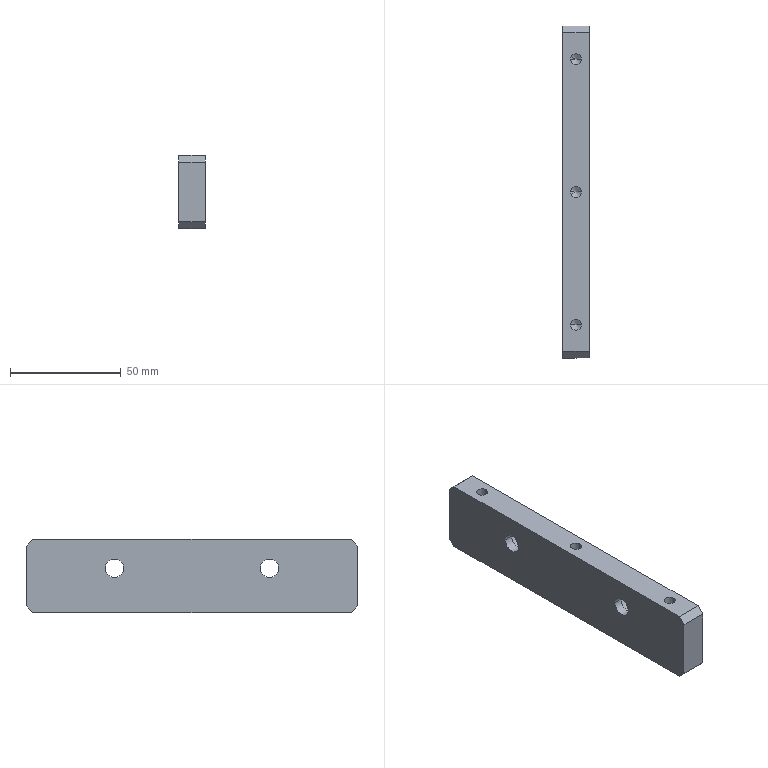Component | SolidWorks | A-C18EjectorMechanismConnectingBlock2-2 | 1 solid | 32 faces | box 12 x 150 x 33 mm | volume 55365 mm3 | cylinder 14 | plane 12 | cone 6 | commonest cylinder face diameters 5 x6 14 x4 8.4 x4
build123d program:
from build123d import *

# Parameters (mm, degrees)
SKETCH1_W                                       = 150
SKETCH1_H                                       = 33
BOSS_EXTRUDE1_DEPTH                             = 12
CHAMFER1_SIZE                                   = 3
M8_HEX_SOCKET_HEAD_CAP_SCREW_CBORE1_D           = 8.4
M8_HEX_SOCKET_HEAD_CAP_SCREW_CBORE1_CBORE_D     = 14
M8_HEX_SOCKET_HEAD_CAP_SCREW_CBORE1_CBORE_DEPTH = 8
M6_TAPPED_HOLE1_D                               = 5
M6_TAPPED_HOLE1_DEPTH                           = 15
M6_TAPPED_HOLE1_TIP                             = 1.502


with BuildPart() as part:
    # Sketch1 → Boss-Extrude1 (new body)
    with BuildSketch(Plane.XY):
        Rectangle(SKETCH1_W, SKETCH1_H)
    extrude(amount=BOSS_EXTRUDE1_DEPTH)

    # Chamfer1
    chamfer1_edges = [part.edges().sort_by_distance(p)[0] for p in [
        (75, -16.5, 6),
        (-75, -16.5, 6),
        (-75, 16.5, 6),
        (75, 16.5, 6),
    ]]
    chamfer(chamfer1_edges, length=CHAMFER1_SIZE)

    # M8 Hex Socket Head Cap Screw CBORE1 (through all)
    with Locations(Plane(origin=(0, 0, 0), x_dir=(-1, 0, 0), z_dir=(0, 0, -1))):
        with Locations((35, -3.5), (-35, -3.5)):
            CounterBoreHole(M8_HEX_SOCKET_HEAD_CAP_SCREW_CBORE1_D / 2, M8_HEX_SOCKET_HEAD_CAP_SCREW_CBORE1_CBORE_D / 2, M8_HEX_SOCKET_HEAD_CAP_SCREW_CBORE1_CBORE_DEPTH)

    # M6 Tapped Hole1
    with Locations(Plane.XZ.offset(16.5)):
        with Locations((-60, 6), (0, 6), (60, 6)):
            Hole(M6_TAPPED_HOLE1_D / 2, depth=M6_TAPPED_HOLE1_DEPTH)
            with Locations((0, 0, -(M6_TAPPED_HOLE1_DEPTH + M6_TAPPED_HOLE1_TIP / 2))):  # 118° drill point
                Cone(0, M6_TAPPED_HOLE1_D / 2, M6_TAPPED_HOLE1_TIP, mode=Mode.SUBTRACT)


solid = part.part

# Placed as in the assembly
solid = solid.moved(Location((-81.181, 22.568, -16.5), (-90, -90, 0)))
STEP:
#1=CARTESIAN_POINT('',(-3.531,-1.474,-0.5906));
#2=VERTEX_POINT('',#1);
#3=CARTESIAN_POINT('',(-3.334,-1.474,-0.5906));
#4=VERTEX_POINT('',#3);
#5=CARTESIAN_POINT('',(-3.432,-1.474,-0.5906));
#6=DIRECTION('',(0.,0.,1.));
#7=DIRECTION('',(1.,0.,0.));
#8=AXIS2_PLACEMENT_3D('',#5,#6,#7);
#9=CIRCLE('',#8,0.09843);
#10=EDGE_CURVE('',#2,#4,#9,.T.);
#11=ORIENTED_EDGE('',*,*,#10,.F.);
#12=CARTESIAN_POINT('',(-3.531,-1.474,-0.));
#13=VERTEX_POINT('',#12);
#14=CARTESIAN_POINT('',(-3.531,-1.474,-0.));
#15=DIRECTION('',(0.,0.,1.));
#16=VECTOR('',#15,39.37);
#17=LINE('',#14,#16);
#18=EDGE_CURVE('',#2,#13,#17,.T.);
#19=ORIENTED_EDGE('',*,*,#18,.T.);
#20=CARTESIAN_POINT('',(-3.334,-1.474,-0.));
#21=VERTEX_POINT('',#20);
#22=CARTESIAN_POINT('',(-3.432,-1.474,-0.));
#23=DIRECTION('',(0.,0.,1.));
#24=DIRECTION('',(1.,0.,0.));
#25=AXIS2_PLACEMENT_3D('',#22,#23,#24);
#26=CIRCLE('',#25,0.09843);
#27=EDGE_CURVE('',#13,#21,#26,.T.);
#28=ORIENTED_EDGE('',*,*,#27,.T.);
#29=CARTESIAN_POINT('',(-3.334,-1.474,-0.));
#30=DIRECTION('',(0.,0.,1.));
#31=VECTOR('',#30,39.37);
#32=LINE('',#29,#31);
#33=EDGE_CURVE('',#4,#21,#32,.T.);
#34=ORIENTED_EDGE('',*,*,#33,.F.);
#35=EDGE_LOOP('',(#11,#19,#28,#34));
#36=FACE_OUTER_BOUND('',#35,.T.);
#37=CARTESIAN_POINT('',(-3.432,-1.474,-0.));
#38=DIRECTION('',(0.,0.,1.));
#39=DIRECTION('',(1.,0.,0.));
#40=AXIS2_PLACEMENT_3D('',#37,#38,#39);
#41=CYLINDRICAL_SURFACE('',#40,0.09843);
#42=ADVANCED_FACE('',(#36),#41,.F.);
#43=CARTESIAN_POINT('',(-3.432,-1.474,-0.6497));
#44=VERTEX_POINT('',#43);
#45=CARTESIAN_POINT('',(-3.334,-1.474,-0.5906));
#46=DIRECTION('',(0.8572,0.,0.515));
#47=VECTOR('',#46,39.37);
#48=LINE('',#45,#47);
#49=EDGE_CURVE('',#44,#4,#48,.T.);
#50=ORIENTED_EDGE('',*,*,#49,.F.);
#51=CARTESIAN_POINT('',(-3.531,-1.474,-0.5906));
#52=DIRECTION('',(-0.8572,0.,0.515));
#53=VECTOR('',#52,39.37);
#54=LINE('',#51,#53);
#55=EDGE_CURVE('',#44,#2,#54,.T.);
#56=ORIENTED_EDGE('',*,*,#55,.T.);
#57=ORIENTED_EDGE('',*,*,#10,.T.);
#58=EDGE_LOOP('',(#50,#56,#57));
#59=FACE_OUTER_BOUND('',#58,.T.);
#60=CARTESIAN_POINT('',(-3.432,-1.474,-0.5906));
#61=DIRECTION('',(0.,0.,1.));
#62=DIRECTION('',(1.,0.,0.));
#63=AXIS2_PLACEMENT_3D('',#60,#61,#62);
#64=CONICAL_SURFACE('',#63,0.09843,1.03);
#65=ADVANCED_FACE('',(#59),#64,.F.);
#66=CARTESIAN_POINT('',(-3.531,0.8885,-0.5906));
#67=VERTEX_POINT('',#66);
#68=CARTESIAN_POINT('',(-3.334,0.8885,-0.5906));
#69=VERTEX_POINT('',#68);
#70=CARTESIAN_POINT('',(-3.432,0.8885,-0.5906));
#71=DIRECTION('',(0.,0.,1.));
#72=DIRECTION('',(1.,0.,0.));
#73=AXIS2_PLACEMENT_3D('',#70,#71,#72);
#74=CIRCLE('',#73,0.09843);
#75=EDGE_CURVE('',#67,#69,#74,.T.);
#76=ORIENTED_EDGE('',*,*,#75,.F.);
#77=CARTESIAN_POINT('',(-3.531,0.8885,-0.));
#78=VERTEX_POINT('',#77);
#79=CARTESIAN_POINT('',(-3.531,0.8885,-0.));
#80=DIRECTION('',(0.,0.,1.));
#81=VECTOR('',#80,39.37);
#82=LINE('',#79,#81);
#83=EDGE_CURVE('',#67,#78,#82,.T.);
#84=ORIENTED_EDGE('',*,*,#83,.T.);
#85=CARTESIAN_POINT('',(-3.334,0.8885,-0.));
#86=VERTEX_POINT('',#85);
#87=CARTESIAN_POINT('',(-3.432,0.8885,-0.));
#88=DIRECTION('',(0.,0.,1.));
#89=DIRECTION('',(1.,0.,0.));
#90=AXIS2_PLACEMENT_3D('',#87,#88,#89);
#91=CIRCLE('',#90,0.09843);
#92=EDGE_CURVE('',#78,#86,#91,.T.);
#93=ORIENTED_EDGE('',*,*,#92,.T.);
#94=CARTESIAN_POINT('',(-3.334,0.8885,-0.));
#95=DIRECTION('',(0.,0.,1.));
#96=VECTOR('',#95,39.37);
#97=LINE('',#94,#96);
#98=EDGE_CURVE('',#69,#86,#97,.T.);
#99=ORIENTED_EDGE('',*,*,#98,.F.);
#100=EDGE_LOOP('',(#76,#84,#93,#99));
#101=FACE_OUTER_BOUND('',#100,.T.);
#102=CARTESIAN_POINT('',(-3.432,0.8885,-0.));
#103=DIRECTION('',(0.,0.,1.));
#104=DIRECTION('',(1.,0.,0.));
#105=AXIS2_PLACEMENT_3D('',#102,#103,#104);
#106=CYLINDRICAL_SURFACE('',#105,0.09843);
#107=ADVANCED_FACE('',(#101),#106,.F.);
#108=CARTESIAN_POINT('',(-3.432,0.8885,-0.6497));
#109=VERTEX_POINT('',#108);
#110=CARTESIAN_POINT('',(-3.334,0.8885,-0.5906));
#111=DIRECTION('',(0.8572,0.,0.515));
#112=VECTOR('',#111,39.37);
#113=LINE('',#110,#112);
#114=EDGE_CURVE('',#109,#69,#113,.T.);
#115=ORIENTED_EDGE('',*,*,#114,.F.);
#116=CARTESIAN_POINT('',(-3.531,0.8885,-0.5906));
#117=DIRECTION('',(-0.8572,0.,0.515));
#118=VECTOR('',#117,39.37);
#119=LINE('',#116,#118);
#120=EDGE_CURVE('',#109,#67,#119,.T.);
#121=ORIENTED_EDGE('',*,*,#120,.T.);
#122=ORIENTED_EDGE('',*,*,#75,.T.);
#123=EDGE_LOOP('',(#115,#121,#122));
#124=FACE_OUTER_BOUND('',#123,.T.);
#125=CARTESIAN_POINT('',(-3.432,0.8885,-0.5906));
#126=DIRECTION('',(0.,0.,1.));
#127=DIRECTION('',(1.,0.,0.));
#128=AXIS2_PLACEMENT_3D('',#125,#126,#127);
#129=CONICAL_SURFACE('',#128,0.09843,1.03);
#130=ADVANCED_FACE('',(#124),#129,.F.);
#131=CARTESIAN_POINT('',(-3.531,3.251,-0.5906));
#132=VERTEX_POINT('',#131);
#133=CARTESIAN_POINT('',(-3.334,3.251,-0.5906));
#134=VERTEX_POINT('',#133);
#135=CARTESIAN_POINT('',(-3.432,3.251,-0.5906));
#136=DIRECTION('',(0.,0.,1.));
#137=DIRECTION('',(1.,0.,0.));
#138=AXIS2_PLACEMENT_3D('',#135,#136,#137);
#139=CIRCLE('',#138,0.09843);
#140=EDGE_CURVE('',#132,#134,#139,.T.);
#141=ORIENTED_EDGE('',*,*,#140,.F.);
#142=CARTESIAN_POINT('',(-3.531,3.251,-0.));
#143=VERTEX_POINT('',#142);
#144=CARTESIAN_POINT('',(-3.531,3.251,-0.));
#145=DIRECTION('',(0.,0.,1.));
#146=VECTOR('',#145,39.37);
#147=LINE('',#144,#146);
#148=EDGE_CURVE('',#132,#143,#147,.T.);
#149=ORIENTED_EDGE('',*,*,#148,.T.);
#150=CARTESIAN_POINT('',(-3.334,3.251,-0.));
#151=VERTEX_POINT('',#150);
#152=CARTESIAN_POINT('',(-3.432,3.251,-0.));
#153=DIRECTION('',(0.,0.,1.));
#154=DIRECTION('',(1.,0.,0.));
#155=AXIS2_PLACEMENT_3D('',#152,#153,#154);
#156=CIRCLE('',#155,0.09843);
#157=EDGE_CURVE('',#143,#151,#156,.T.);
#158=ORIENTED_EDGE('',*,*,#157,.T.);
#159=CARTESIAN_POINT('',(-3.334,3.251,-0.));
#160=DIRECTION('',(0.,0.,1.));
#161=VECTOR('',#160,39.37);
#162=LINE('',#159,#161);
#163=EDGE_CURVE('',#134,#151,#162,.T.);
#164=ORIENTED_EDGE('',*,*,#163,.F.);
#165=EDGE_LOOP('',(#141,#149,#158,#164));
#166=FACE_OUTER_BOUND('',#165,.T.);
#167=CARTESIAN_POINT('',(-3.432,3.251,-0.));
#168=DIRECTION('',(0.,0.,1.));
#169=DIRECTION('',(1.,0.,0.));
#170=AXIS2_PLACEMENT_3D('',#167,#168,#169);
#171=CYLINDRICAL_SURFACE('',#170,0.09843);
#172=ADVANCED_FACE('',(#166),#171,.F.);
#173=CARTESIAN_POINT('',(-3.432,3.251,-0.6497));
#174=VERTEX_POINT('',#173);
#175=CARTESIAN_POINT('',(-3.334,3.251,-0.5906));
#176=DIRECTION('',(0.8572,0.,0.515));
#177=VECTOR('',#176,39.37);
#178=LINE('',#175,#177);
#179=EDGE_CURVE('',#174,#134,#178,.T.);
#180=ORIENTED_EDGE('',*,*,#179,.F.);
#181=CARTESIAN_POINT('',(-3.531,3.251,-0.5906));
#182=DIRECTION('',(-0.8572,0.,0.515));
#183=VECTOR('',#182,39.37);
#184=LINE('',#181,#183);
#185=EDGE_CURVE('',#174,#132,#184,.T.);
#186=ORIENTED_EDGE('',*,*,#185,.T.);
#187=ORIENTED_EDGE('',*,*,#140,.T.);
#188=EDGE_LOOP('',(#180,#186,#187));
#189=FACE_OUTER_BOUND('',#188,.T.);
#190=CARTESIAN_POINT('',(-3.432,3.251,-0.5906));
#191=DIRECTION('',(0.,0.,1.));
#192=DIRECTION('',(1.,0.,0.));
#193=AXIS2_PLACEMENT_3D('',#190,#191,#192);
#194=CONICAL_SURFACE('',#193,0.09843,1.03);
#195=ADVANCED_FACE('',(#189),#194,.F.);
#196=CARTESIAN_POINT('',(-3.511,-0.2138,-0.5118));
#197=VERTEX_POINT('',#196);
#198=CARTESIAN_POINT('',(-3.511,-0.765,-0.5118));
#199=VERTEX_POINT('',#198);
#200=CARTESIAN_POINT('',(-3.511,-0.4894,-0.5118));
#201=DIRECTION('',(1.,0.,0.));
#202=DIRECTION('',(0.,-1.,0.));
#203=AXIS2_PLACEMENT_3D('',#200,#201,#202);
#204=CIRCLE('',#203,0.2756);
#205=EDGE_CURVE('',#197,#199,#204,.T.);
#206=ORIENTED_EDGE('',*,*,#205,.F.);
#207=CARTESIAN_POINT('',(-3.196,-0.2138,-0.5118));
#208=VERTEX_POINT('',#207);
#209=CARTESIAN_POINT('',(-3.196,-0.2138,-0.5118));
#210=DIRECTION('',(1.,0.,0.));
#211=VECTOR('',#210,39.37);
#212=LINE('',#209,#211);
#213=EDGE_CURVE('',#197,#208,#212,.T.);
#214=ORIENTED_EDGE('',*,*,#213,.T.);
#215=CARTESIAN_POINT('',(-3.196,-0.765,-0.5118));
#216=VERTEX_POINT('',#215);
#217=CARTESIAN_POINT('',(-3.196,-0.4894,-0.5118));
#218=DIRECTION('',(1.,0.,0.));
#219=DIRECTION('',(0.,-1.,0.));
#220=AXIS2_PLACEMENT_3D('',#217,#218,#219);
#221=CIRCLE('',#220,0.2756);
#222=EDGE_CURVE('',#208,#216,#221,.T.);
#223=ORIENTED_EDGE('',*,*,#222,.T.);
#224=CARTESIAN_POINT('',(-3.196,-0.765,-0.5118));
#225=DIRECTION('',(1.,0.,0.));
#226=VECTOR('',#225,39.37);
#227=LINE('',#224,#226);
#228=EDGE_CURVE('',#199,#216,#227,.T.);
#229=ORIENTED_EDGE('',*,*,#228,.F.);
#230=EDGE_LOOP('',(#206,#214,#223,#229));
#231=FACE_OUTER_BOUND('',#230,.T.);
#232=CARTESIAN_POINT('',(-3.196,-0.4894,-0.5118));
#233=DIRECTION('',(1.,0.,0.));
#234=DIRECTION('',(0.,-1.,0.));
#235=AXIS2_PLACEMENT_3D('',#232,#233,#234);
#236=CYLINDRICAL_SURFACE('',#235,0.2756);
#237=ADVANCED_FACE('',(#231),#236,.F.);
#238=CARTESIAN_POINT('',(-3.669,-0.3241,-0.5118));
#239=VERTEX_POINT('',#238);
#240=CARTESIAN_POINT('',(-3.669,-0.6548,-0.5118));
#241=VERTEX_POINT('',#240);
#242=CARTESIAN_POINT('',(-3.669,-0.4894,-0.5118));
#243=DIRECTION('',(1.,0.,0.));
#244=DIRECTION('',(0.,-1.,0.));
#245=AXIS2_PLACEMENT_3D('',#242,#243,#244);
#246=CIRCLE('',#245,0.1654);
#247=EDGE_CURVE('',#239,#241,#246,.T.);
#248=ORIENTED_EDGE('',*,*,#247,.F.);
#249=CARTESIAN_POINT('',(-3.511,-0.3241,-0.5118));
#250=VERTEX_POINT('',#249);
#251=CARTESIAN_POINT('',(-3.196,-0.3241,-0.5118));
#252=DIRECTION('',(1.,0.,0.));
#253=VECTOR('',#252,39.37);
#254=LINE('',#251,#253);
#255=EDGE_CURVE('',#239,#250,#254,.T.);
#256=ORIENTED_EDGE('',*,*,#255,.T.);
#257=CARTESIAN_POINT('',(-3.511,-0.6548,-0.5118));
#258=VERTEX_POINT('',#257);
#259=CARTESIAN_POINT('',(-3.511,-0.4894,-0.5118));
#260=DIRECTION('',(1.,0.,0.));
#261=DIRECTION('',(0.,-1.,0.));
#262=AXIS2_PLACEMENT_3D('',#259,#260,#261);
#263=CIRCLE('',#262,0.1654);
#264=EDGE_CURVE('',#250,#258,#263,.T.);
#265=ORIENTED_EDGE('',*,*,#264,.T.);
#266=CARTESIAN_POINT('',(-3.196,-0.6548,-0.5118));
#267=DIRECTION('',(1.,0.,0.));
#268=VECTOR('',#267,39.37);
#269=LINE('',#266,#268);
#270=EDGE_CURVE('',#241,#258,#269,.T.);
#271=ORIENTED_EDGE('',*,*,#270,.F.);
#272=EDGE_LOOP('',(#248,#256,#265,#271));
#273=FACE_OUTER_BOUND('',#272,.T.);
#274=CARTESIAN_POINT('',(-3.196,-0.4894,-0.5118));
#275=DIRECTION('',(1.,0.,0.));
#276=DIRECTION('',(0.,-1.,0.));
#277=AXIS2_PLACEMENT_3D('',#274,#275,#276);
#278=CYLINDRICAL_SURFACE('',#277,0.1654);
#279=ADVANCED_FACE('',(#273),#278,.F.);
#280=CARTESIAN_POINT('',(-3.511,2.542,-0.5118));
#281=VERTEX_POINT('',#280);
#282=CARTESIAN_POINT('',(-3.511,1.991,-0.5118));
#283=VERTEX_POINT('',#282);
#284=CARTESIAN_POINT('',(-3.511,2.266,-0.5118));
#285=DIRECTION('',(1.,0.,0.));
#286=DIRECTION('',(0.,-1.,0.));
#287=AXIS2_PLACEMENT_3D('',#284,#285,#286);
#288=CIRCLE('',#287,0.2756);
#289=EDGE_CURVE('',#281,#283,#288,.T.);
#290=ORIENTED_EDGE('',*,*,#289,.F.);
#291=CARTESIAN_POINT('',(-3.196,2.542,-0.5118));
#292=VERTEX_POINT('',#291);
#293=CARTESIAN_POINT('',(-3.196,2.542,-0.5118));
#294=DIRECTION('',(1.,0.,0.));
#295=VECTOR('',#294,39.37);
#296=LINE('',#293,#295);
#297=EDGE_CURVE('',#281,#292,#296,.T.);
#298=ORIENTED_EDGE('',*,*,#297,.T.);
#299=CARTESIAN_POINT('',(-3.196,1.991,-0.5118));
#300=VERTEX_POINT('',#299);
#301=CARTESIAN_POINT('',(-3.196,2.266,-0.5118));
#302=DIRECTION('',(1.,0.,0.));
#303=DIRECTION('',(0.,-1.,0.));
#304=AXIS2_PLACEMENT_3D('',#301,#302,#303);
#305=CIRCLE('',#304,0.2756);
#306=EDGE_CURVE('',#292,#300,#305,.T.);
#307=ORIENTED_EDGE('',*,*,#306,.T.);
#308=CARTESIAN_POINT('',(-3.196,1.991,-0.5118));
#309=DIRECTION('',(1.,0.,0.));
#310=VECTOR('',#309,39.37);
#311=LINE('',#308,#310);
#312=EDGE_CURVE('',#283,#300,#311,.T.);
#313=ORIENTED_EDGE('',*,*,#312,.F.);
#314=EDGE_LOOP('',(#290,#298,#307,#313));
#315=FACE_OUTER_BOUND('',#314,.T.);
#316=CARTESIAN_POINT('',(-3.196,2.266,-0.5118));
#317=DIRECTION('',(1.,0.,0.));
#318=DIRECTION('',(0.,-1.,0.));
#319=AXIS2_PLACEMENT_3D('',#316,#317,#318);
#320=CYLINDRICAL_SURFACE('',#319,0.2756);
#321=ADVANCED_FACE('',(#315),#320,.F.);
#322=CARTESIAN_POINT('',(-3.669,2.432,-0.5118));
#323=VERTEX_POINT('',#322);
#324=CARTESIAN_POINT('',(-3.669,2.101,-0.5118));
#325=VERTEX_POINT('',#324);
#326=CARTESIAN_POINT('',(-3.669,2.266,-0.5118));
#327=DIRECTION('',(1.,0.,0.));
#328=DIRECTION('',(0.,-1.,0.));
#329=AXIS2_PLACEMENT_3D('',#326,#327,#328);
#330=CIRCLE('',#329,0.1654);
#331=EDGE_CURVE('',#323,#325,#330,.T.);
#332=ORIENTED_EDGE('',*,*,#331,.F.);
#333=CARTESIAN_POINT('',(-3.511,2.432,-0.5118));
#334=VERTEX_POINT('',#333);
#335=CARTESIAN_POINT('',(-3.196,2.432,-0.5118));
#336=DIRECTION('',(1.,0.,0.));
#337=VECTOR('',#336,39.37);
#338=LINE('',#335,#337);
#339=EDGE_CURVE('',#323,#334,#338,.T.);
#340=ORIENTED_EDGE('',*,*,#339,.T.);
#341=CARTESIAN_POINT('',(-3.511,2.101,-0.5118));
#342=VERTEX_POINT('',#341);
#343=CARTESIAN_POINT('',(-3.511,2.266,-0.5118));
#344=DIRECTION('',(1.,0.,0.));
#345=DIRECTION('',(0.,-1.,0.));
#346=AXIS2_PLACEMENT_3D('',#343,#344,#345);
#347=CIRCLE('',#346,0.1654);
#348=EDGE_CURVE('',#334,#342,#347,.T.);
#349=ORIENTED_EDGE('',*,*,#348,.T.);
#350=CARTESIAN_POINT('',(-3.196,2.101,-0.5118));
#351=DIRECTION('',(1.,0.,0.));
#352=VECTOR('',#351,39.37);
#353=LINE('',#350,#352);
#354=EDGE_CURVE('',#325,#342,#353,.T.);
#355=ORIENTED_EDGE('',*,*,#354,.F.);
#356=EDGE_LOOP('',(#332,#340,#349,#355));
#357=FACE_OUTER_BOUND('',#356,.T.);
#358=CARTESIAN_POINT('',(-3.196,2.266,-0.5118));
#359=DIRECTION('',(1.,0.,0.));
#360=DIRECTION('',(0.,-1.,0.));
#361=AXIS2_PLACEMENT_3D('',#358,#359,#360);
#362=CYLINDRICAL_SURFACE('',#361,0.1654);
#363=ADVANCED_FACE('',(#357),#362,.F.);
#364=CARTESIAN_POINT('',(-3.196,3.841,-0.1181));
#365=VERTEX_POINT('',#364);
#366=CARTESIAN_POINT('',(-3.196,3.841,-1.181));
#367=VERTEX_POINT('',#366);
#368=CARTESIAN_POINT('',(-3.196,3.841,-1.299));
#369=DIRECTION('',(0.,0.,-1.));
#370=VECTOR('',#369,39.37);
#371=LINE('',#368,#370);
#372=EDGE_CURVE('',#365,#367,#371,.T.);
#373=ORIENTED_EDGE('',*,*,#372,.T.);
#374=CARTESIAN_POINT('',(-3.669,3.841,-1.181));
#375=VERTEX_POINT('',#374);
#376=CARTESIAN_POINT('',(-3.669,3.841,-1.181));
#377=DIRECTION('',(-1.,0.,0.));
#378=VECTOR('',#377,39.37);
#379=LINE('',#376,#378);
#380=EDGE_CURVE('',#367,#375,#379,.T.);
#381=ORIENTED_EDGE('',*,*,#380,.T.);
#382=CARTESIAN_POINT('',(-3.669,3.841,-0.1181));
#383=VERTEX_POINT('',#382);
#384=CARTESIAN_POINT('',(-3.669,3.841,-1.299));
#385=DIRECTION('',(0.,0.,-1.));
#386=VECTOR('',#385,39.37);
#387=LINE('',#384,#386);
#388=EDGE_CURVE('',#383,#375,#387,.T.);
#389=ORIENTED_EDGE('',*,*,#388,.F.);
#390=CARTESIAN_POINT('',(-3.669,3.841,-0.1181));
#391=DIRECTION('',(1.,0.,0.));
#392=VECTOR('',#391,39.37);
#393=LINE('',#390,#392);
#394=EDGE_CURVE('',#383,#365,#393,.T.);
#395=ORIENTED_EDGE('',*,*,#394,.T.);
#396=EDGE_LOOP('',(#373,#381,#389,#395));
#397=FACE_OUTER_BOUND('',#396,.T.);
#398=CARTESIAN_POINT('',(-3.669,3.841,-1.299));
#399=DIRECTION('',(0.,-1.,0.));
#400=DIRECTION('',(-1.,0.,0.));
#401=AXIS2_PLACEMENT_3D('',#398,#399,#400);
#402=PLANE('',#401);
#403=ADVANCED_FACE('',(#397),#402,.F.);
#404=CARTESIAN_POINT('',(-3.669,3.723,-1.299));
#405=VERTEX_POINT('',#404);
#406=CARTESIAN_POINT('',(-3.669,-1.946,-1.299));
#407=VERTEX_POINT('',#406);
#408=CARTESIAN_POINT('',(-3.669,-2.064,-1.299));
#409=DIRECTION('',(0.,-1.,0.));
#410=VECTOR('',#409,39.37);
#411=LINE('',#408,#410);
#412=EDGE_CURVE('',#405,#407,#411,.T.);
#413=ORIENTED_EDGE('',*,*,#412,.F.);
#414=CARTESIAN_POINT('',(-3.196,3.723,-1.299));
#415=VERTEX_POINT('',#414);
#416=CARTESIAN_POINT('',(-3.669,3.723,-1.299));
#417=DIRECTION('',(1.,0.,0.));
#418=VECTOR('',#417,39.37);
#419=LINE('',#416,#418);
#420=EDGE_CURVE('',#405,#415,#419,.T.);
#421=ORIENTED_EDGE('',*,*,#420,.T.);
#422=CARTESIAN_POINT('',(-3.196,-1.946,-1.299));
#423=VERTEX_POINT('',#422);
#424=CARTESIAN_POINT('',(-3.196,-2.064,-1.299));
#425=DIRECTION('',(0.,-1.,0.));
#426=VECTOR('',#425,39.37);
#427=LINE('',#424,#426);
#428=EDGE_CURVE('',#415,#423,#427,.T.);
#429=ORIENTED_EDGE('',*,*,#428,.T.);
#430=CARTESIAN_POINT('',(-3.669,-1.946,-1.299));
#431=DIRECTION('',(-1.,0.,0.));
#432=VECTOR('',#431,39.37);
#433=LINE('',#430,#432);
#434=EDGE_CURVE('',#423,#407,#433,.T.);
#435=ORIENTED_EDGE('',*,*,#434,.T.);
#436=EDGE_LOOP('',(#413,#421,#429,#435));
#437=FACE_OUTER_BOUND('',#436,.T.);
#438=CARTESIAN_POINT('',(-3.669,-2.064,-1.299));
#439=DIRECTION('',(0.,0.,1.));
#440=DIRECTION('',(1.,0.,0.));
#441=AXIS2_PLACEMENT_3D('',#438,#439,#440);
#442=PLANE('',#441);
#443=ADVANCED_FACE('',(#437),#442,.F.);
#444=CARTESIAN_POINT('',(-3.669,-2.064,-1.181));
#445=VERTEX_POINT('',#444);
#446=CARTESIAN_POINT('',(-3.669,-2.064,-0.1181));
#447=VERTEX_POINT('',#446);
#448=CARTESIAN_POINT('',(-3.669,-2.064,-1.299));
#449=DIRECTION('',(0.,0.,1.));
#450=VECTOR('',#449,39.37);
#451=LINE('',#448,#450);
#452=EDGE_CURVE('',#445,#447,#451,.T.);
#453=ORIENTED_EDGE('',*,*,#452,.F.);
#454=CARTESIAN_POINT('',(-3.196,-2.064,-1.181));
#455=VERTEX_POINT('',#454);
#456=CARTESIAN_POINT('',(-3.669,-2.064,-1.181));
#457=DIRECTION('',(1.,0.,0.));
#458=VECTOR('',#457,39.37);
#459=LINE('',#456,#458);
#460=EDGE_CURVE('',#445,#455,#459,.T.);
#461=ORIENTED_EDGE('',*,*,#460,.T.);
#462=CARTESIAN_POINT('',(-3.196,-2.064,-0.1181));
#463=VERTEX_POINT('',#462);
#464=CARTESIAN_POINT('',(-3.196,-2.064,-1.299));
#465=DIRECTION('',(0.,0.,1.));
#466=VECTOR('',#465,39.37);
#467=LINE('',#464,#466);
#468=EDGE_CURVE('',#455,#463,#467,.T.);
#469=ORIENTED_EDGE('',*,*,#468,.T.);
#470=CARTESIAN_POINT('',(-3.669,-2.064,-0.1181));
#471=DIRECTION('',(-1.,0.,0.));
#472=VECTOR('',#471,39.37);
#473=LINE('',#470,#472);
#474=EDGE_CURVE('',#463,#447,#473,.T.);
#475=ORIENTED_EDGE('',*,*,#474,.T.);
#476=EDGE_LOOP('',(#453,#461,#469,#475));
#477=FACE_OUTER_BOUND('',#476,.T.);
#478=CARTESIAN_POINT('',(-3.669,-2.064,-1.299));
#479=DIRECTION('',(0.,1.,0.));
#480=DIRECTION('',(1.,0.,0.));
#481=AXIS2_PLACEMENT_3D('',#478,#479,#480);
#482=PLANE('',#481);
#483=ADVANCED_FACE('',(#477),#482,.F.);
#484=CARTESIAN_POINT('',(-3.432,-1.474,-0.));
#485=DIRECTION('',(0.,0.,1.));
#486=DIRECTION('',(1.,0.,0.));
#487=AXIS2_PLACEMENT_3D('',#484,#485,#486);
#488=CIRCLE('',#487,0.09843);
#489=EDGE_CURVE('',#21,#13,#488,.T.);
#490=ORIENTED_EDGE('',*,*,#489,.F.);
#491=ORIENTED_EDGE('',*,*,#27,.F.);
#492=EDGE_LOOP('',(#490,#491));
#493=FACE_BOUND('',#492,.T.);
#494=CARTESIAN_POINT('',(-3.432,0.8885,-0.));
#495=DIRECTION('',(0.,0.,1.));
#496=DIRECTION('',(1.,0.,0.));
#497=AXIS2_PLACEMENT_3D('',#494,#495,#496);
#498=CIRCLE('',#497,0.09843);
#499=EDGE_CURVE('',#86,#78,#498,.T.);
#500=ORIENTED_EDGE('',*,*,#499,.F.);
#501=ORIENTED_EDGE('',*,*,#92,.F.);
#502=EDGE_LOOP('',(#500,#501));
#503=FACE_BOUND('',#502,.T.);
#504=CARTESIAN_POINT('',(-3.432,3.251,-0.));
#505=DIRECTION('',(0.,0.,1.));
#506=DIRECTION('',(1.,0.,0.));
#507=AXIS2_PLACEMENT_3D('',#504,#505,#506);
#508=CIRCLE('',#507,0.09843);
#509=EDGE_CURVE('',#151,#143,#508,.T.);
#510=ORIENTED_EDGE('',*,*,#509,.F.);
#511=ORIENTED_EDGE('',*,*,#157,.F.);
#512=EDGE_LOOP('',(#510,#511));
#513=FACE_BOUND('',#512,.T.);
#514=CARTESIAN_POINT('',(-3.196,-1.946,-0.));
#515=VERTEX_POINT('',#514);
#516=CARTESIAN_POINT('',(-3.196,3.723,-0.));
#517=VERTEX_POINT('',#516);
#518=CARTESIAN_POINT('',(-3.196,-2.064,-0.));
#519=DIRECTION('',(0.,1.,0.));
#520=VECTOR('',#519,39.37);
#521=LINE('',#518,#520);
#522=EDGE_CURVE('',#515,#517,#521,.T.);
#523=ORIENTED_EDGE('',*,*,#522,.T.);
#524=CARTESIAN_POINT('',(-3.669,3.723,-0.));
#525=VERTEX_POINT('',#524);
#526=CARTESIAN_POINT('',(-3.669,3.723,-0.));
#527=DIRECTION('',(-1.,0.,0.));
#528=VECTOR('',#527,39.37);
#529=LINE('',#526,#528);
#530=EDGE_CURVE('',#517,#525,#529,.T.);
#531=ORIENTED_EDGE('',*,*,#530,.T.);
#532=CARTESIAN_POINT('',(-3.669,-1.946,-0.));
#533=VERTEX_POINT('',#532);
#534=CARTESIAN_POINT('',(-3.669,-2.064,-0.));
#535=DIRECTION('',(0.,1.,0.));
#536=VECTOR('',#535,39.37);
#537=LINE('',#534,#536);
#538=EDGE_CURVE('',#533,#525,#537,.T.);
#539=ORIENTED_EDGE('',*,*,#538,.F.);
#540=CARTESIAN_POINT('',(-3.669,-1.946,-0.));
#541=DIRECTION('',(1.,0.,0.));
#542=VECTOR('',#541,39.37);
#543=LINE('',#540,#542);
#544=EDGE_CURVE('',#533,#515,#543,.T.);
#545=ORIENTED_EDGE('',*,*,#544,.T.);
#546=EDGE_LOOP('',(#523,#531,#539,#545));
#547=FACE_OUTER_BOUND('',#546,.T.);
#548=CARTESIAN_POINT('',(-3.669,-2.064,-0.));
#549=DIRECTION('',(0.,0.,-1.));
#550=DIRECTION('',(-1.,0.,0.));
#551=AXIS2_PLACEMENT_3D('',#548,#549,#550);
#552=PLANE('',#551);
#553=ADVANCED_FACE('',(#493,#503,#513,#547),#552,.F.);
#554=CARTESIAN_POINT('',(-3.669,-0.4894,-0.5118));
#555=DIRECTION('',(1.,0.,0.));
#556=DIRECTION('',(0.,-1.,0.));
#557=AXIS2_PLACEMENT_3D('',#554,#555,#556);
#558=CIRCLE('',#557,0.1654);
#559=EDGE_CURVE('',#241,#239,#558,.T.);
#560=ORIENTED_EDGE('',*,*,#559,.T.);
#561=ORIENTED_EDGE('',*,*,#247,.T.);
#562=EDGE_LOOP('',(#560,#561));
#563=FACE_BOUND('',#562,.T.);
#564=CARTESIAN_POINT('',(-3.669,2.266,-0.5118));
#565=DIRECTION('',(1.,0.,0.));
#566=DIRECTION('',(0.,-1.,0.));
#567=AXIS2_PLACEMENT_3D('',#564,#565,#566);
#568=CIRCLE('',#567,0.1654);
#569=EDGE_CURVE('',#325,#323,#568,.T.);
#570=ORIENTED_EDGE('',*,*,#569,.T.);
#571=ORIENTED_EDGE('',*,*,#331,.T.);
#572=EDGE_LOOP('',(#570,#571));
#573=FACE_BOUND('',#572,.T.);
#574=ORIENTED_EDGE('',*,*,#388,.T.);
#575=CARTESIAN_POINT('',(-3.669,4.432,-0.5906));
#576=DIRECTION('',(0.,-0.7071,-0.7071));
#577=VECTOR('',#576,39.37);
#578=LINE('',#575,#577);
#579=EDGE_CURVE('',#375,#405,#578,.T.);
#580=ORIENTED_EDGE('',*,*,#579,.T.);
#581=ORIENTED_EDGE('',*,*,#412,.T.);
#582=CARTESIAN_POINT('',(-3.669,0.298,-3.543));
#583=DIRECTION('',(0.,-0.7071,0.7071));
#584=VECTOR('',#583,39.37);
#585=LINE('',#582,#584);
#586=EDGE_CURVE('',#407,#445,#585,.T.);
#587=ORIENTED_EDGE('',*,*,#586,.T.);
#588=ORIENTED_EDGE('',*,*,#452,.T.);
#589=CARTESIAN_POINT('',(-3.669,0.9476,2.894));
#590=DIRECTION('',(0.,0.7071,0.7071));
#591=VECTOR('',#590,39.37);
#592=LINE('',#589,#591);
#593=EDGE_CURVE('',#447,#533,#592,.T.);
#594=ORIENTED_EDGE('',*,*,#593,.T.);
#595=ORIENTED_EDGE('',*,*,#538,.T.);
#596=CARTESIAN_POINT('',(-3.669,3.782,-0.05906));
#597=DIRECTION('',(0.,0.7071,-0.7071));
#598=VECTOR('',#597,39.37);
#599=LINE('',#596,#598);
#600=EDGE_CURVE('',#525,#383,#599,.T.);
#601=ORIENTED_EDGE('',*,*,#600,.T.);
#602=EDGE_LOOP('',(#574,#580,#581,#587,#588,#594,#595,#601));
#603=FACE_OUTER_BOUND('',#602,.T.);
#604=CARTESIAN_POINT('',(-3.669,3.841,-0.));
#605=DIRECTION('',(-1.,0.,0.));
#606=DIRECTION('',(0.,1.,0.));
#607=AXIS2_PLACEMENT_3D('',#604,#605,#606);
#608=PLANE('',#607);
#609=ADVANCED_FACE('',(#563,#573,#603),#608,.T.);
#610=CARTESIAN_POINT('',(-3.196,-0.4894,-0.5118));
#611=DIRECTION('',(1.,0.,0.));
#612=DIRECTION('',(0.,-1.,0.));
#613=AXIS2_PLACEMENT_3D('',#610,#611,#612);
#614=CIRCLE('',#613,0.2756);
#615=EDGE_CURVE('',#216,#208,#614,.T.);
#616=ORIENTED_EDGE('',*,*,#615,.F.);
#617=ORIENTED_EDGE('',*,*,#222,.F.);
#618=EDGE_LOOP('',(#616,#617));
#619=FACE_BOUND('',#618,.T.);
#620=CARTESIAN_POINT('',(-3.196,2.266,-0.5118));
#621=DIRECTION('',(1.,0.,0.));
#622=DIRECTION('',(0.,-1.,0.));
#623=AXIS2_PLACEMENT_3D('',#620,#621,#622);
#624=CIRCLE('',#623,0.2756);
#625=EDGE_CURVE('',#300,#292,#624,.T.);
#626=ORIENTED_EDGE('',*,*,#625,.F.);
#627=ORIENTED_EDGE('',*,*,#306,.F.);
#628=EDGE_LOOP('',(#626,#627));
#629=FACE_BOUND('',#628,.T.);
#630=ORIENTED_EDGE('',*,*,#428,.F.);
#631=CARTESIAN_POINT('',(-3.196,3.723,-1.299));
#632=DIRECTION('',(0.,0.7071,0.7071));
#633=VECTOR('',#632,39.37);
#634=LINE('',#631,#633);
#635=EDGE_CURVE('',#415,#367,#634,.T.);
#636=ORIENTED_EDGE('',*,*,#635,.T.);
#637=ORIENTED_EDGE('',*,*,#372,.F.);
#638=CARTESIAN_POINT('',(-3.196,3.841,-0.1181));
#639=DIRECTION('',(0.,-0.7071,0.7071));
#640=VECTOR('',#639,39.37);
#641=LINE('',#638,#640);
#642=EDGE_CURVE('',#365,#517,#641,.T.);
#643=ORIENTED_EDGE('',*,*,#642,.T.);
#644=ORIENTED_EDGE('',*,*,#522,.F.);
#645=CARTESIAN_POINT('',(-3.196,-1.946,-0.));
#646=DIRECTION('',(0.,-0.7071,-0.7071));
#647=VECTOR('',#646,39.37);
#648=LINE('',#645,#647);
#649=EDGE_CURVE('',#515,#463,#648,.T.);
#650=ORIENTED_EDGE('',*,*,#649,.T.);
#651=ORIENTED_EDGE('',*,*,#468,.F.);
#652=CARTESIAN_POINT('',(-3.196,-2.064,-1.181));
#653=DIRECTION('',(0.,0.7071,-0.7071));
#654=VECTOR('',#653,39.37);
#655=LINE('',#652,#654);
#656=EDGE_CURVE('',#455,#423,#655,.T.);
#657=ORIENTED_EDGE('',*,*,#656,.T.);
#658=EDGE_LOOP('',(#630,#636,#637,#643,#644,#650,#651,#657));
#659=FACE_OUTER_BOUND('',#658,.T.);
#660=CARTESIAN_POINT('',(-3.196,3.841,-0.));
#661=DIRECTION('',(-1.,0.,0.));
#662=DIRECTION('',(0.,1.,0.));
#663=AXIS2_PLACEMENT_3D('',#660,#661,#662);
#664=PLANE('',#663);
#665=ADVANCED_FACE('',(#619,#629,#659),#664,.F.);
#666=ORIENTED_EDGE('',*,*,#579,.F.);
#667=ORIENTED_EDGE('',*,*,#380,.F.);
#668=ORIENTED_EDGE('',*,*,#635,.F.);
#669=ORIENTED_EDGE('',*,*,#420,.F.);
#670=EDGE_LOOP('',(#666,#667,#668,#669));
#671=FACE_OUTER_BOUND('',#670,.T.);
#672=CARTESIAN_POINT('',(-3.669,3.723,-1.299));
#673=DIRECTION('',(0.,-0.7071,0.7071));
#674=DIRECTION('',(0.,0.7071,0.7071));
#675=AXIS2_PLACEMENT_3D('',#672,#673,#674);
#676=PLANE('',#675);
#677=ADVANCED_FACE('',(#671),#676,.F.);
#678=ORIENTED_EDGE('',*,*,#600,.F.);
#679=ORIENTED_EDGE('',*,*,#530,.F.);
#680=ORIENTED_EDGE('',*,*,#642,.F.);
#681=ORIENTED_EDGE('',*,*,#394,.F.);
#682=EDGE_LOOP('',(#678,#679,#680,#681));
#683=FACE_OUTER_BOUND('',#682,.T.);
#684=CARTESIAN_POINT('',(-3.669,3.841,-0.1181));
#685=DIRECTION('',(0.,-0.7071,-0.7071));
#686=DIRECTION('',(0.,-0.7071,0.7071));
#687=AXIS2_PLACEMENT_3D('',#684,#685,#686);
#688=PLANE('',#687);
#689=ADVANCED_FACE('',(#683),#688,.F.);
#690=ORIENTED_EDGE('',*,*,#586,.F.);
#691=ORIENTED_EDGE('',*,*,#434,.F.);
#692=ORIENTED_EDGE('',*,*,#656,.F.);
#693=ORIENTED_EDGE('',*,*,#460,.F.);
#694=EDGE_LOOP('',(#690,#691,#692,#693));
#695=FACE_OUTER_BOUND('',#694,.T.);
#696=CARTESIAN_POINT('',(-3.669,-2.064,-1.181));
#697=DIRECTION('',(0.,0.7071,0.7071));
#698=DIRECTION('',(0.,0.7071,-0.7071));
#699=AXIS2_PLACEMENT_3D('',#696,#697,#698);
#700=PLANE('',#699);
#701=ADVANCED_FACE('',(#695),#700,.F.);
#702=ORIENTED_EDGE('',*,*,#593,.F.);
#703=ORIENTED_EDGE('',*,*,#474,.F.);
#704=ORIENTED_EDGE('',*,*,#649,.F.);
#705=ORIENTED_EDGE('',*,*,#544,.F.);
#706=EDGE_LOOP('',(#702,#703,#704,#705));
#707=FACE_OUTER_BOUND('',#706,.T.);
#708=CARTESIAN_POINT('',(-3.669,-1.946,-0.));
#709=DIRECTION('',(0.,0.7071,-0.7071));
#710=DIRECTION('',(0.,-0.7071,-0.7071));
#711=AXIS2_PLACEMENT_3D('',#708,#709,#710);
#712=PLANE('',#711);
#713=ADVANCED_FACE('',(#707),#712,.F.);
#714=ORIENTED_EDGE('',*,*,#339,.F.);
#715=ORIENTED_EDGE('',*,*,#569,.F.);
#716=ORIENTED_EDGE('',*,*,#354,.T.);
#717=CARTESIAN_POINT('',(-3.511,2.266,-0.5118));
#718=DIRECTION('',(1.,0.,0.));
#719=DIRECTION('',(0.,-1.,0.));
#720=AXIS2_PLACEMENT_3D('',#717,#718,#719);
#721=CIRCLE('',#720,0.1654);
#722=EDGE_CURVE('',#342,#334,#721,.T.);
#723=ORIENTED_EDGE('',*,*,#722,.T.);
#724=EDGE_LOOP('',(#714,#715,#716,#723));
#725=FACE_OUTER_BOUND('',#724,.T.);
#726=CARTESIAN_POINT('',(-3.196,2.266,-0.5118));
#727=DIRECTION('',(1.,0.,0.));
#728=DIRECTION('',(0.,-1.,0.));
#729=AXIS2_PLACEMENT_3D('',#726,#727,#728);
#730=CYLINDRICAL_SURFACE('',#729,0.1654);
#731=ADVANCED_FACE('',(#725),#730,.F.);
#732=ORIENTED_EDGE('',*,*,#722,.F.);
#733=ORIENTED_EDGE('',*,*,#348,.F.);
#734=EDGE_LOOP('',(#732,#733));
#735=FACE_BOUND('',#734,.T.);
#736=CARTESIAN_POINT('',(-3.511,2.266,-0.5118));
#737=DIRECTION('',(1.,0.,0.));
#738=DIRECTION('',(0.,-1.,0.));
#739=AXIS2_PLACEMENT_3D('',#736,#737,#738);
#740=CIRCLE('',#739,0.2756);
#741=EDGE_CURVE('',#283,#281,#740,.T.);
#742=ORIENTED_EDGE('',*,*,#741,.T.);
#743=ORIENTED_EDGE('',*,*,#289,.T.);
#744=EDGE_LOOP('',(#742,#743));
#745=FACE_OUTER_BOUND('',#744,.T.);
#746=CARTESIAN_POINT('',(-3.511,2.432,-0.5118));
#747=DIRECTION('',(-1.,0.,0.));
#748=DIRECTION('',(0.,1.,0.));
#749=AXIS2_PLACEMENT_3D('',#746,#747,#748);
#750=PLANE('',#749);
#751=ADVANCED_FACE('',(#735,#745),#750,.F.);
#752=ORIENTED_EDGE('',*,*,#297,.F.);
#753=ORIENTED_EDGE('',*,*,#741,.F.);
#754=ORIENTED_EDGE('',*,*,#312,.T.);
#755=ORIENTED_EDGE('',*,*,#625,.T.);
#756=EDGE_LOOP('',(#752,#753,#754,#755));
#757=FACE_OUTER_BOUND('',#756,.T.);
#758=CARTESIAN_POINT('',(-3.196,2.266,-0.5118));
#759=DIRECTION('',(1.,0.,0.));
#760=DIRECTION('',(0.,-1.,0.));
#761=AXIS2_PLACEMENT_3D('',#758,#759,#760);
#762=CYLINDRICAL_SURFACE('',#761,0.2756);
#763=ADVANCED_FACE('',(#757),#762,.F.);
#764=ORIENTED_EDGE('',*,*,#255,.F.);
#765=ORIENTED_EDGE('',*,*,#559,.F.);
#766=ORIENTED_EDGE('',*,*,#270,.T.);
#767=CARTESIAN_POINT('',(-3.511,-0.4894,-0.5118));
#768=DIRECTION('',(1.,0.,0.));
#769=DIRECTION('',(0.,-1.,0.));
#770=AXIS2_PLACEMENT_3D('',#767,#768,#769);
#771=CIRCLE('',#770,0.1654);
#772=EDGE_CURVE('',#258,#250,#771,.T.);
#773=ORIENTED_EDGE('',*,*,#772,.T.);
#774=EDGE_LOOP('',(#764,#765,#766,#773));
#775=FACE_OUTER_BOUND('',#774,.T.);
#776=CARTESIAN_POINT('',(-3.196,-0.4894,-0.5118));
#777=DIRECTION('',(1.,0.,0.));
#778=DIRECTION('',(0.,-1.,0.));
#779=AXIS2_PLACEMENT_3D('',#776,#777,#778);
#780=CYLINDRICAL_SURFACE('',#779,0.1654);
#781=ADVANCED_FACE('',(#775),#780,.F.);
#782=ORIENTED_EDGE('',*,*,#772,.F.);
#783=ORIENTED_EDGE('',*,*,#264,.F.);
#784=EDGE_LOOP('',(#782,#783));
#785=FACE_BOUND('',#784,.T.);
#786=CARTESIAN_POINT('',(-3.511,-0.4894,-0.5118));
#787=DIRECTION('',(1.,0.,0.));
#788=DIRECTION('',(0.,-1.,0.));
#789=AXIS2_PLACEMENT_3D('',#786,#787,#788);
#790=CIRCLE('',#789,0.2756);
#791=EDGE_CURVE('',#199,#197,#790,.T.);
#792=ORIENTED_EDGE('',*,*,#791,.T.);
#793=ORIENTED_EDGE('',*,*,#205,.T.);
#794=EDGE_LOOP('',(#792,#793));
#795=FACE_OUTER_BOUND('',#794,.T.);
#796=CARTESIAN_POINT('',(-3.511,-0.3241,-0.5118));
#797=DIRECTION('',(-1.,0.,0.));
#798=DIRECTION('',(0.,1.,0.));
#799=AXIS2_PLACEMENT_3D('',#796,#797,#798);
#800=PLANE('',#799);
#801=ADVANCED_FACE('',(#785,#795),#800,.F.);
#802=ORIENTED_EDGE('',*,*,#213,.F.);
#803=ORIENTED_EDGE('',*,*,#791,.F.);
#804=ORIENTED_EDGE('',*,*,#228,.T.);
#805=ORIENTED_EDGE('',*,*,#615,.T.);
#806=EDGE_LOOP('',(#802,#803,#804,#805));
#807=FACE_OUTER_BOUND('',#806,.T.);
#808=CARTESIAN_POINT('',(-3.196,-0.4894,-0.5118));
#809=DIRECTION('',(1.,0.,0.));
#810=DIRECTION('',(0.,-1.,0.));
#811=AXIS2_PLACEMENT_3D('',#808,#809,#810);
#812=CYLINDRICAL_SURFACE('',#811,0.2756);
#813=ADVANCED_FACE('',(#807),#812,.F.);
#814=ORIENTED_EDGE('',*,*,#185,.F.);
#815=ORIENTED_EDGE('',*,*,#179,.T.);
#816=CARTESIAN_POINT('',(-3.432,3.251,-0.5906));
#817=DIRECTION('',(0.,0.,1.));
#818=DIRECTION('',(1.,0.,0.));
#819=AXIS2_PLACEMENT_3D('',#816,#817,#818);
#820=CIRCLE('',#819,0.09843);
#821=EDGE_CURVE('',#134,#132,#820,.T.);
#822=ORIENTED_EDGE('',*,*,#821,.T.);
#823=EDGE_LOOP('',(#814,#815,#822));
#824=FACE_OUTER_BOUND('',#823,.T.);
#825=CARTESIAN_POINT('',(-3.432,3.251,-0.5906));
#826=DIRECTION('',(0.,0.,1.));
#827=DIRECTION('',(1.,0.,0.));
#828=AXIS2_PLACEMENT_3D('',#825,#826,#827);
#829=CONICAL_SURFACE('',#828,0.09843,1.03);
#830=ADVANCED_FACE('',(#824),#829,.F.);
#831=ORIENTED_EDGE('',*,*,#148,.F.);
#832=ORIENTED_EDGE('',*,*,#821,.F.);
#833=ORIENTED_EDGE('',*,*,#163,.T.);
#834=ORIENTED_EDGE('',*,*,#509,.T.);
#835=EDGE_LOOP('',(#831,#832,#833,#834));
#836=FACE_OUTER_BOUND('',#835,.T.);
#837=CARTESIAN_POINT('',(-3.432,3.251,-0.));
#838=DIRECTION('',(0.,0.,1.));
#839=DIRECTION('',(1.,0.,0.));
#840=AXIS2_PLACEMENT_3D('',#837,#838,#839);
#841=CYLINDRICAL_SURFACE('',#840,0.09843);
#842=ADVANCED_FACE('',(#836),#841,.F.);
#843=ORIENTED_EDGE('',*,*,#120,.F.);
#844=ORIENTED_EDGE('',*,*,#114,.T.);
#845=CARTESIAN_POINT('',(-3.432,0.8885,-0.5906));
#846=DIRECTION('',(0.,0.,1.));
#847=DIRECTION('',(1.,0.,0.));
#848=AXIS2_PLACEMENT_3D('',#845,#846,#847);
#849=CIRCLE('',#848,0.09843);
#850=EDGE_CURVE('',#69,#67,#849,.T.);
#851=ORIENTED_EDGE('',*,*,#850,.T.);
#852=EDGE_LOOP('',(#843,#844,#851));
#853=FACE_OUTER_BOUND('',#852,.T.);
#854=CARTESIAN_POINT('',(-3.432,0.8885,-0.5906));
#855=DIRECTION('',(0.,0.,1.));
#856=DIRECTION('',(1.,0.,0.));
#857=AXIS2_PLACEMENT_3D('',#854,#855,#856);
#858=CONICAL_SURFACE('',#857,0.09843,1.03);
#859=ADVANCED_FACE('',(#853),#858,.F.);
#860=ORIENTED_EDGE('',*,*,#83,.F.);
#861=ORIENTED_EDGE('',*,*,#850,.F.);
#862=ORIENTED_EDGE('',*,*,#98,.T.);
#863=ORIENTED_EDGE('',*,*,#499,.T.);
#864=EDGE_LOOP('',(#860,#861,#862,#863));
#865=FACE_OUTER_BOUND('',#864,.T.);
#866=CARTESIAN_POINT('',(-3.432,0.8885,-0.));
#867=DIRECTION('',(0.,0.,1.));
#868=DIRECTION('',(1.,0.,0.));
#869=AXIS2_PLACEMENT_3D('',#866,#867,#868);
#870=CYLINDRICAL_SURFACE('',#869,0.09843);
#871=ADVANCED_FACE('',(#865),#870,.F.);
#872=ORIENTED_EDGE('',*,*,#55,.F.);
#873=ORIENTED_EDGE('',*,*,#49,.T.);
#874=CARTESIAN_POINT('',(-3.432,-1.474,-0.5906));
#875=DIRECTION('',(0.,0.,1.));
#876=DIRECTION('',(1.,0.,0.));
#877=AXIS2_PLACEMENT_3D('',#874,#875,#876);
#878=CIRCLE('',#877,0.09843);
#879=EDGE_CURVE('',#4,#2,#878,.T.);
#880=ORIENTED_EDGE('',*,*,#879,.T.);
#881=EDGE_LOOP('',(#872,#873,#880));
#882=FACE_OUTER_BOUND('',#881,.T.);
#883=CARTESIAN_POINT('',(-3.432,-1.474,-0.5906));
#884=DIRECTION('',(0.,0.,1.));
#885=DIRECTION('',(1.,0.,0.));
#886=AXIS2_PLACEMENT_3D('',#883,#884,#885);
#887=CONICAL_SURFACE('',#886,0.09843,1.03);
#888=ADVANCED_FACE('',(#882),#887,.F.);
#889=ORIENTED_EDGE('',*,*,#18,.F.);
#890=ORIENTED_EDGE('',*,*,#879,.F.);
#891=ORIENTED_EDGE('',*,*,#33,.T.);
#892=ORIENTED_EDGE('',*,*,#489,.T.);
#893=EDGE_LOOP('',(#889,#890,#891,#892));
#894=FACE_OUTER_BOUND('',#893,.T.);
#895=CARTESIAN_POINT('',(-3.432,-1.474,-0.));
#896=DIRECTION('',(0.,0.,1.));
#897=DIRECTION('',(1.,0.,0.));
#898=AXIS2_PLACEMENT_3D('',#895,#896,#897);
#899=CYLINDRICAL_SURFACE('',#898,0.09843);
#900=ADVANCED_FACE('',(#894),#899,.F.);
#901=CLOSED_SHELL('',(#42,#65,#107,#130,#172,#195,#237,#279,#321,#363,#403,#443,#483,#553,#609,#665,#677,#689,#701,#713,#731,#751,#763,#781,#801,#813,#830,#842,#859,#871,#888,#900));
#902=MANIFOLD_SOLID_BREP('',#901);
#903=CARTESIAN_POINT('',(0.,0.,0.));
#904=DIRECTION('',(0.,0.,1.));
#905=DIRECTION('',(1.,0.,0.));
#906=AXIS2_PLACEMENT_3D('',#903,#904,#905);
#907=(LENGTH_UNIT()NAMED_UNIT(*)SI_UNIT($,.METRE.));
#908=LENGTH_MEASURE_WITH_UNIT(LENGTH_MEASURE(0.0254),#907);
#909=DIMENSIONAL_EXPONENTS(1.,0.,0.,0.,0.,0.,0.);
#910=(CONVERSION_BASED_UNIT('',#908)LENGTH_UNIT()NAMED_UNIT(#909));
#911=UNCERTAINTY_MEASURE_WITH_UNIT(LENGTH_MEASURE(0.00001),#910,'','');
#912=(NAMED_UNIT(*)PLANE_ANGLE_UNIT()SI_UNIT($,.RADIAN.));
#913=(NAMED_UNIT(*)SI_UNIT($,.STERADIAN.)SOLID_ANGLE_UNIT());
#914=(GEOMETRIC_REPRESENTATION_CONTEXT(3)GLOBAL_UNCERTAINTY_ASSIGNED_CONTEXT((#911))GLOBAL_UNIT_ASSIGNED_CONTEXT((#910,#912,#913))REPRESENTATION_CONTEXT('',''));
#915=ADVANCED_BREP_SHAPE_REPRESENTATION('',(#902,#906),#914);
#916=COLOUR_RGB('',0.7922,0.8196,0.9333);
#917=FILL_AREA_STYLE_COLOUR('',#916);
#918=FILL_AREA_STYLE('',(#917));
#919=SURFACE_STYLE_FILL_AREA(#918);
#920=SURFACE_SIDE_STYLE('',(#919));
#921=SURFACE_STYLE_USAGE(.BOTH.,#920);
#922=PRESENTATION_STYLE_ASSIGNMENT((#921));
#923=STYLED_ITEM('',(#922),#902);
#924=PRESENTATION_LAYER_ASSIGNMENT('','',(#923));
#925=(LENGTH_UNIT()NAMED_UNIT(*)SI_UNIT($,.METRE.));
#926=LENGTH_MEASURE_WITH_UNIT(LENGTH_MEASURE(0.0254),#925);
#927=DIMENSIONAL_EXPONENTS(1.,0.,0.,0.,0.,0.,0.);
#928=(CONVERSION_BASED_UNIT('',#926)LENGTH_UNIT()NAMED_UNIT(#927));
#929=UNCERTAINTY_MEASURE_WITH_UNIT(LENGTH_MEASURE(0.00001),#928,'','');
#930=(NAMED_UNIT(*)PLANE_ANGLE_UNIT()SI_UNIT($,.RADIAN.));
#931=(NAMED_UNIT(*)SI_UNIT($,.STERADIAN.)SOLID_ANGLE_UNIT());
#932=(GEOMETRIC_REPRESENTATION_CONTEXT(3)GLOBAL_UNCERTAINTY_ASSIGNED_CONTEXT((#929))GLOBAL_UNIT_ASSIGNED_CONTEXT((#928,#930,#931))REPRESENTATION_CONTEXT('',''));
#933=MECHANICAL_DESIGN_GEOMETRIC_PRESENTATION_REPRESENTATION('',(#923),#932);